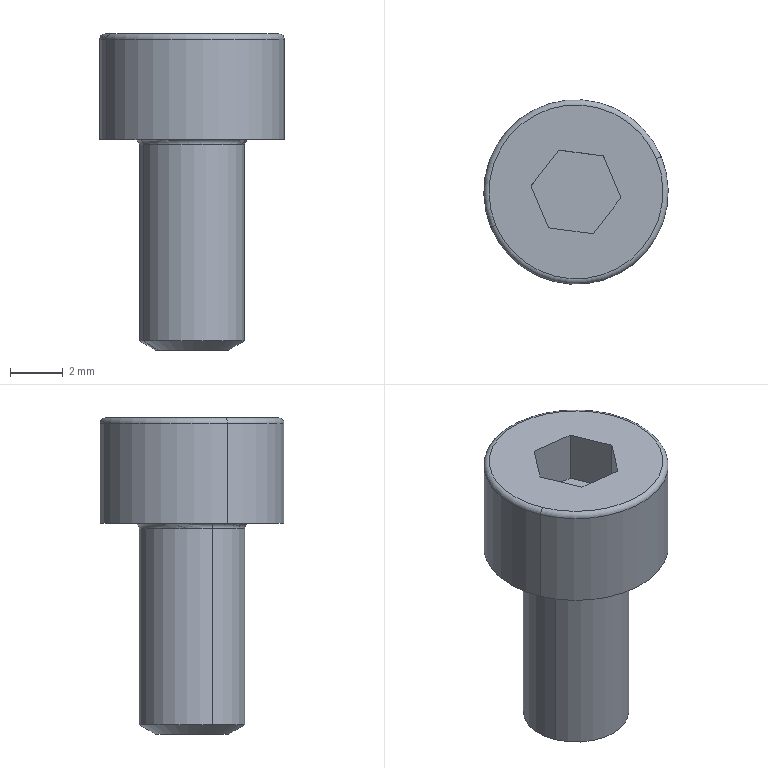Component | NX | GB_T_70_1_HEX_SOCKET_CAP_SCREW_M4X8_3 | 1 solid | 20 faces | volume 238 mm3 | plane 10 | torus 4 | cylinder 4 | cone 2 | commonest cylinder face diameters 7 x2 4 x2